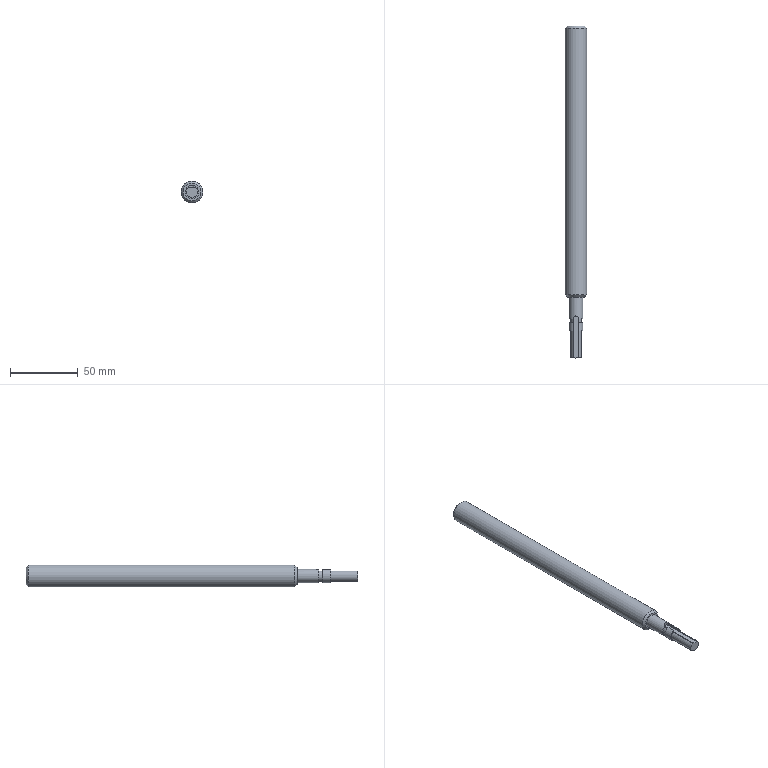Component | NX | WORK_TABLE_SCREW | 1 solid | 17 faces | volume 42870 mm3 | plane 9 | cylinder 6 | cone 2 | commonest cylinder face diameters 10 x2 8 x2 3.5 x1 16 x1